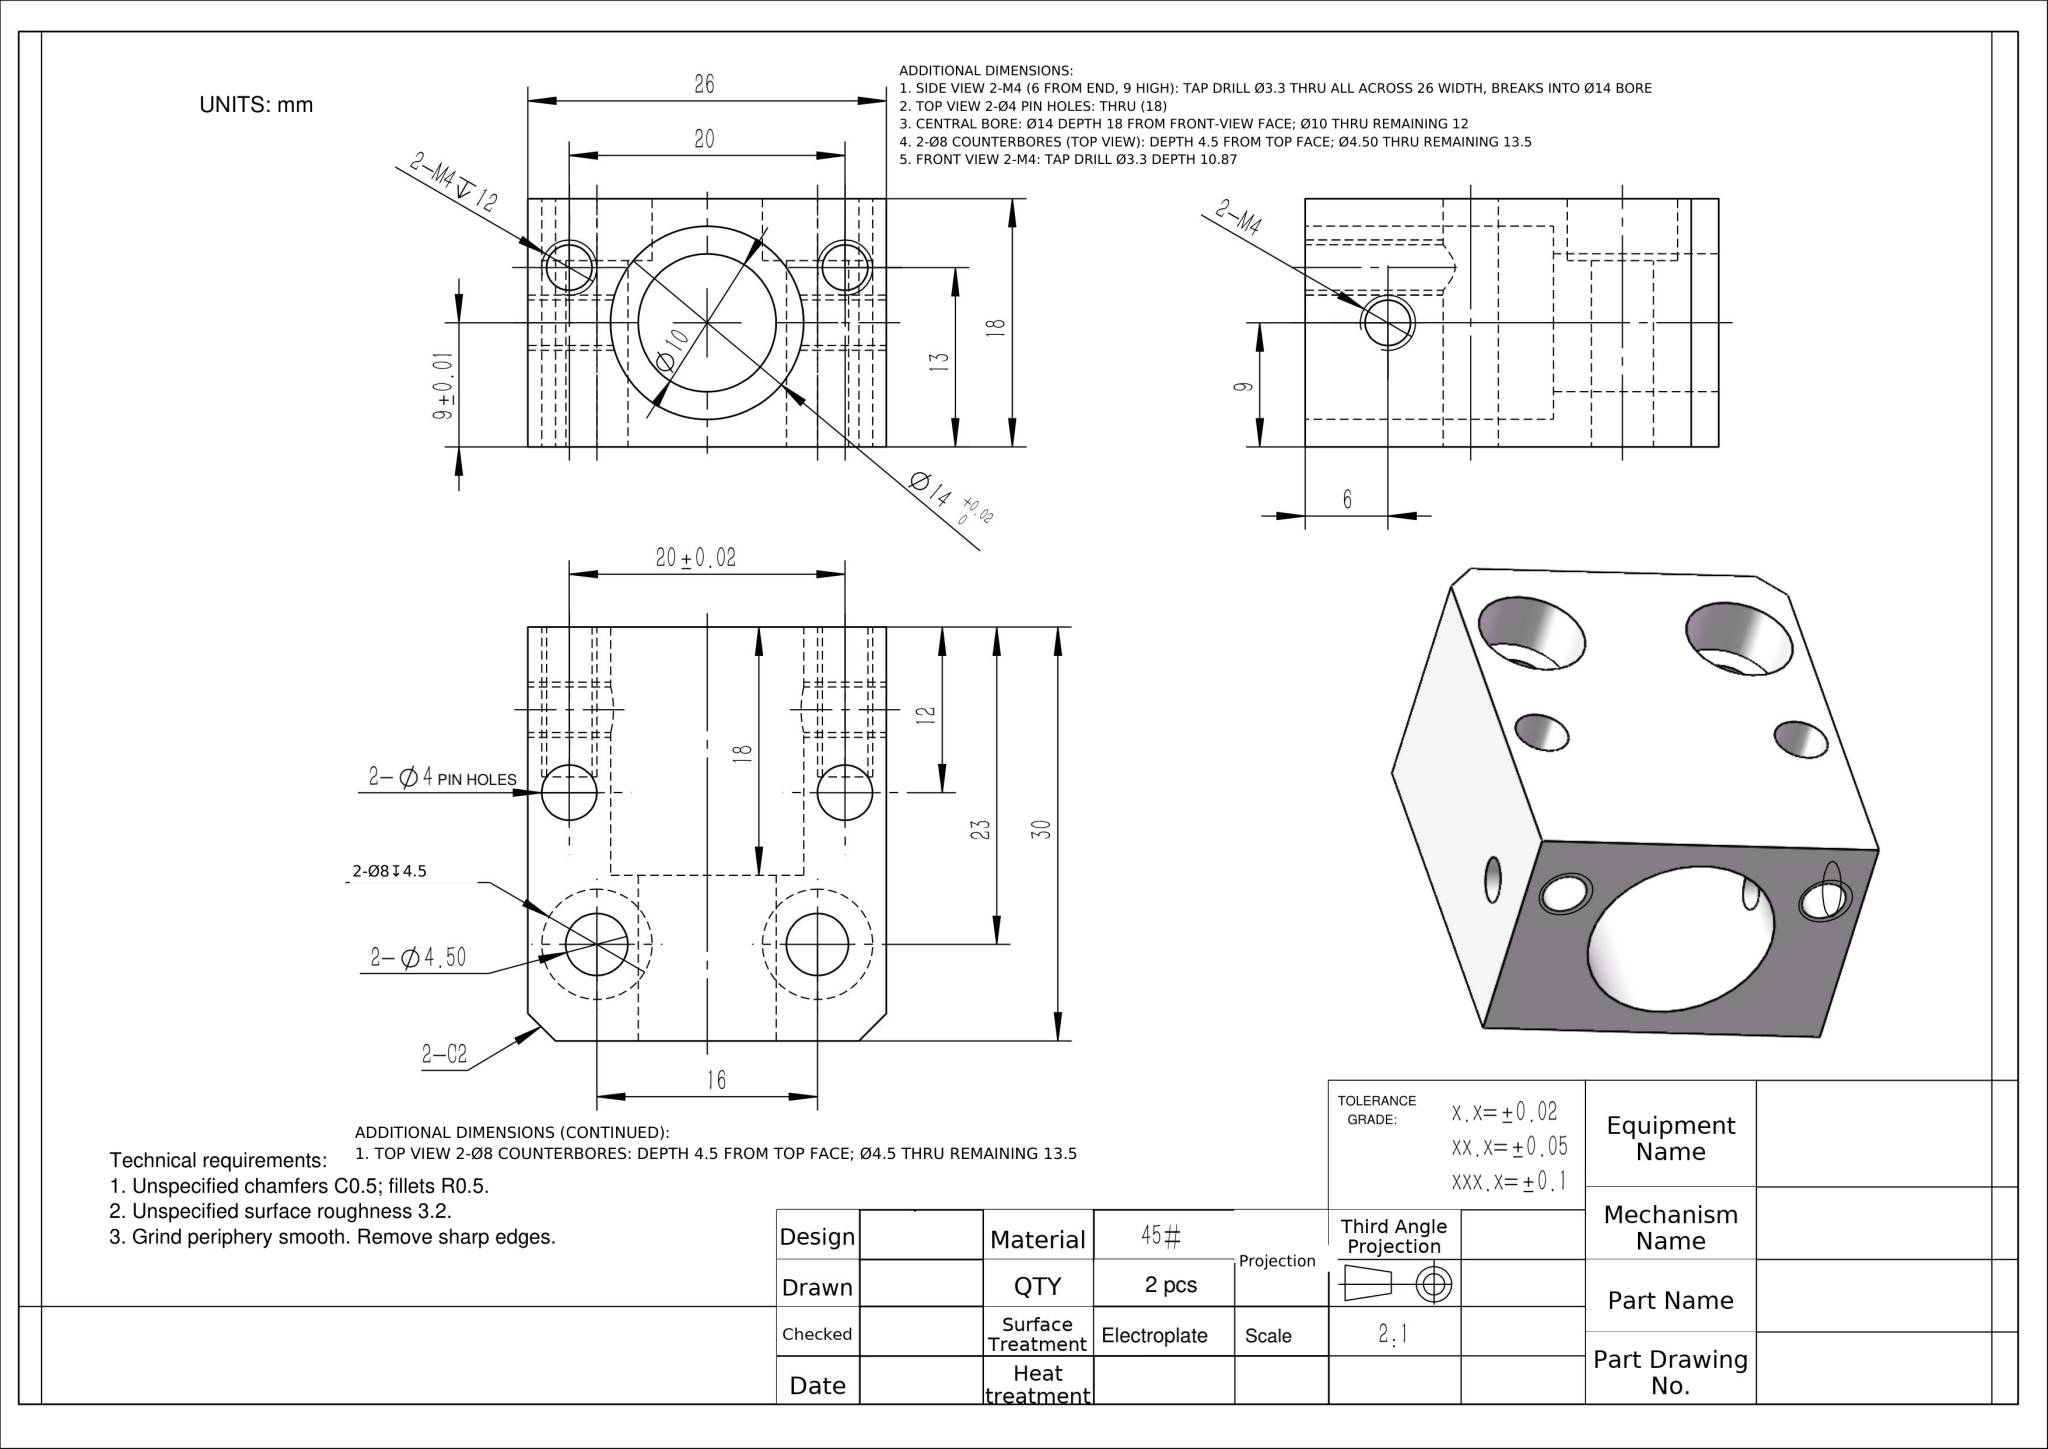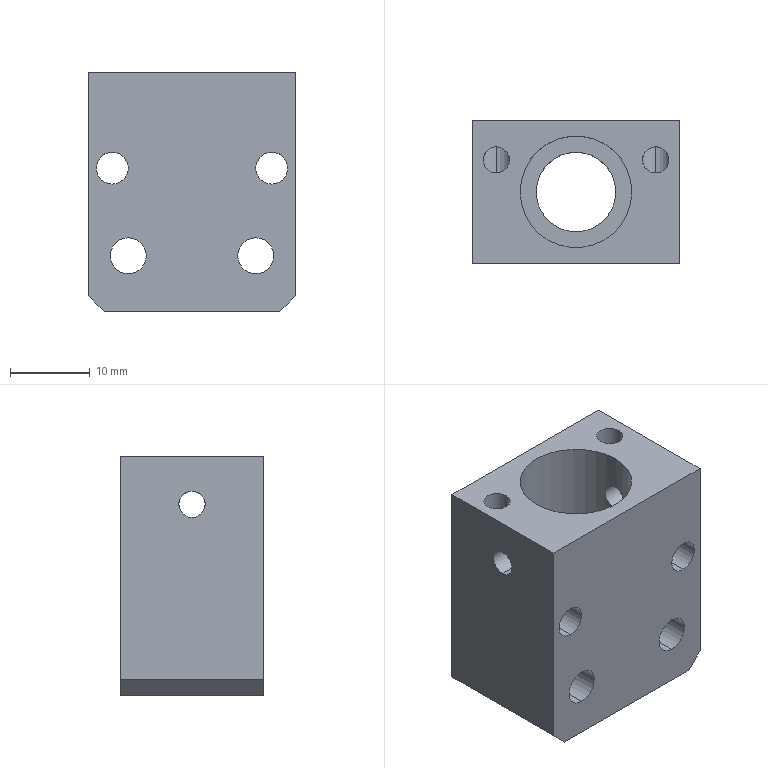Part | NX | mm | 1 solid | 35 faces | box 26 x 18 x 30 mm | volume 8643 mm3 | cylinder 24 | plane 11 | commonest cylinder face diameters 3.3 x8 8 x4 4 x4 4.5 x4 10 x2 14 x2